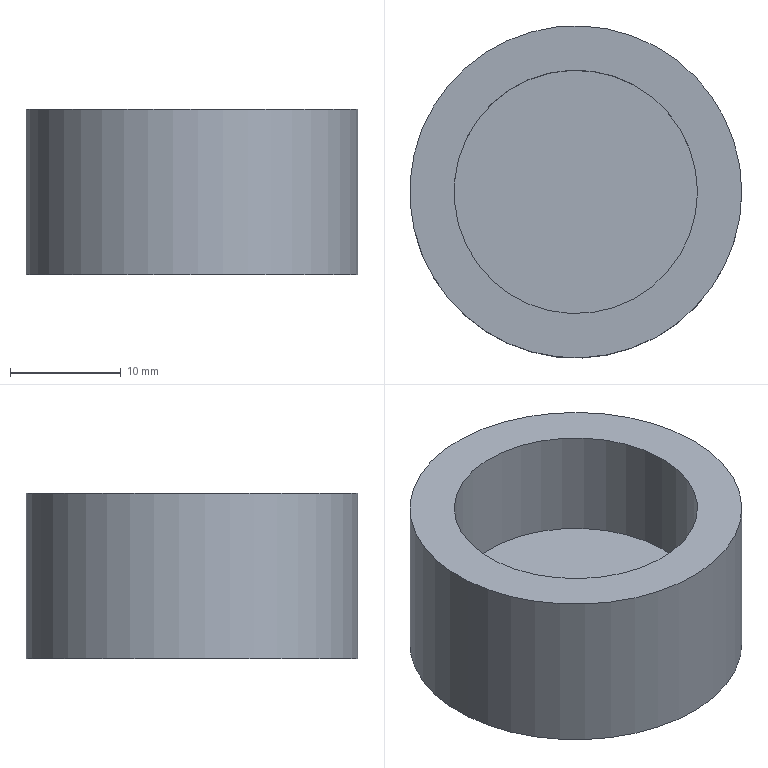Component | NX | CUP | 1 solid | 5 faces | box 30 x 30 x 15 mm | volume 6802 mm3 | plane 3 | cylinder 2 | commonest cylinder face diameters 30 x1 22 x1
STEP:
#1=CARTESIAN_POINT('',(0.,0.,0.));
#2=DIRECTION('',(0.,0.,1.));
#3=DIRECTION('',(1.,0.,0.));
#4=AXIS2_PLACEMENT_3D('',#1,#2,#3);
#5=CARTESIAN_POINT('',(23.5,0.,-28.5));
#6=VERTEX_POINT('',#5);
#7=CARTESIAN_POINT('',(12.5,0.,-28.5));
#8=DIRECTION('',(0.,0.,-1.));
#9=DIRECTION('',(1.,0.,0.));
#10=AXIS2_PLACEMENT_3D('',#7,#8,#9);
#11=CIRCLE('',#10,11.);
#12=CARTESIAN_POINT('',(12.5,0.,-28.5));
#13=DIRECTION('',(0.,0.,1.));
#14=DIRECTION('',(1.,0.,0.));
#15=AXIS2_PLACEMENT_3D('',#12,#13,#14);
#16=PLANE('',#15);
#17=CARTESIAN_POINT('',(11.,0.));
#18=CARTESIAN_POINT('',(11.,-19.053));
#19=CARTESIAN_POINT('',(-5.5,-9.526));
#20=CARTESIAN_POINT('',(-22.,-0.));
#21=CARTESIAN_POINT('',(-5.5,9.526));
#22=CARTESIAN_POINT('',(11.,19.053));
#23=CARTESIAN_POINT('',(11.,0.));
#24=(BOUNDED_CURVE()B_SPLINE_CURVE(2,(#17,#18,#19,#20,#21,#22,#23),.UNSPECIFIED.,.T.,.F.)B_SPLINE_CURVE_WITH_KNOTS((1,2,2,2,2,1),(-2.094,0.,2.094,4.189,6.283,8.378),.UNSPECIFIED.)CURVE()GEOMETRIC_REPRESENTATION_ITEM()RATIONAL_B_SPLINE_CURVE((1.,0.5,1.,0.5,1.,0.5,1.))REPRESENTATION_ITEM(''));
#25=(GEOMETRIC_REPRESENTATION_CONTEXT(2)PARAMETRIC_REPRESENTATION_CONTEXT()REPRESENTATION_CONTEXT('',''));
#26=DEFINITIONAL_REPRESENTATION('',(#24),#25);
#27=PCURVE('',#16,#26);
#28=CARTESIAN_POINT('',(12.5,0.,-38.5));
#29=DIRECTION('',(0.,0.,1.));
#30=DIRECTION('',(1.,0.,0.));
#31=AXIS2_PLACEMENT_3D('',#28,#29,#30);
#32=CYLINDRICAL_SURFACE('',#31,11.);
#33=CARTESIAN_POINT('',(6.283,10.));
#34=DIRECTION('',(-1.,0.));
#35=VECTOR('',#34,1.);
#36=LINE('',#33,#35);
#37=(GEOMETRIC_REPRESENTATION_CONTEXT(2)PARAMETRIC_REPRESENTATION_CONTEXT()REPRESENTATION_CONTEXT('',''));
#38=DEFINITIONAL_REPRESENTATION('',(#36),#37);
#39=PCURVE('',#32,#38);
#40=SURFACE_CURVE('',#11,(#27,#39),.PCURVE_S1.);
#41=EDGE_CURVE('',#6,#6,#40,.T.);
#42=ORIENTED_EDGE('',*,*,#41,.T.);
#43=EDGE_LOOP('',(#42));
#44=FACE_BOUND('',#43,.T.);
#45=CARTESIAN_POINT('',(27.5,0.,-28.5));
#46=VERTEX_POINT('',#45);
#47=CARTESIAN_POINT('',(12.5,0.,-28.5));
#48=DIRECTION('',(0.,0.,-1.));
#49=DIRECTION('',(1.,0.,0.));
#50=AXIS2_PLACEMENT_3D('',#47,#48,#49);
#51=CIRCLE('',#50,15.);
#52=CARTESIAN_POINT('',(15.,0.));
#53=CARTESIAN_POINT('',(15.,-25.981));
#54=CARTESIAN_POINT('',(-7.5,-12.99));
#55=CARTESIAN_POINT('',(-30.,-0.));
#56=CARTESIAN_POINT('',(-7.5,12.99));
#57=CARTESIAN_POINT('',(15.,25.981));
#58=CARTESIAN_POINT('',(15.,0.));
#59=(BOUNDED_CURVE()B_SPLINE_CURVE(2,(#52,#53,#54,#55,#56,#57,#58),.UNSPECIFIED.,.T.,.F.)B_SPLINE_CURVE_WITH_KNOTS((1,2,2,2,2,1),(-2.094,0.,2.094,4.189,6.283,8.378),.UNSPECIFIED.)CURVE()GEOMETRIC_REPRESENTATION_ITEM()RATIONAL_B_SPLINE_CURVE((1.,0.5,1.,0.5,1.,0.5,1.))REPRESENTATION_ITEM(''));
#60=(GEOMETRIC_REPRESENTATION_CONTEXT(2)PARAMETRIC_REPRESENTATION_CONTEXT()REPRESENTATION_CONTEXT('',''));
#61=DEFINITIONAL_REPRESENTATION('',(#59),#60);
#62=PCURVE('',#16,#61);
#63=CARTESIAN_POINT('',(12.5,0.,-43.5));
#64=DIRECTION('',(0.,0.,1.));
#65=DIRECTION('',(1.,0.,0.));
#66=AXIS2_PLACEMENT_3D('',#63,#64,#65);
#67=CYLINDRICAL_SURFACE('',#66,15.);
#68=CARTESIAN_POINT('',(6.283,15.));
#69=DIRECTION('',(-1.,0.));
#70=VECTOR('',#69,1.);
#71=LINE('',#68,#70);
#72=(GEOMETRIC_REPRESENTATION_CONTEXT(2)PARAMETRIC_REPRESENTATION_CONTEXT()REPRESENTATION_CONTEXT('',''));
#73=DEFINITIONAL_REPRESENTATION('',(#71),#72);
#74=PCURVE('',#67,#73);
#75=SURFACE_CURVE('',#51,(#62,#74),.PCURVE_S1.);
#76=EDGE_CURVE('',#46,#46,#75,.T.);
#77=ORIENTED_EDGE('',*,*,#76,.F.);
#78=EDGE_LOOP('',(#77));
#79=FACE_BOUND('',#78,.T.);
#80=ADVANCED_FACE('',(#44,#79),#16,.T.);
#81=CARTESIAN_POINT('',(27.5,0.,-43.5));
#82=VERTEX_POINT('',#81);
#83=CARTESIAN_POINT('',(12.5,0.,-43.5));
#84=DIRECTION('',(0.,0.,1.));
#85=DIRECTION('',(1.,0.,0.));
#86=AXIS2_PLACEMENT_3D('',#83,#84,#85);
#87=CIRCLE('',#86,15.);
#88=CARTESIAN_POINT('',(12.5,0.,-43.5));
#89=DIRECTION('',(0.,0.,-1.));
#90=DIRECTION('',(-1.,0.,0.));
#91=AXIS2_PLACEMENT_3D('',#88,#89,#90);
#92=PLANE('',#91);
#93=CARTESIAN_POINT('',(-15.,0.));
#94=CARTESIAN_POINT('',(-15.,25.981));
#95=CARTESIAN_POINT('',(7.5,12.99));
#96=CARTESIAN_POINT('',(30.,0.));
#97=CARTESIAN_POINT('',(7.5,-12.99));
#98=CARTESIAN_POINT('',(-15.,-25.981));
#99=CARTESIAN_POINT('',(-15.,0.));
#100=(BOUNDED_CURVE()B_SPLINE_CURVE(2,(#93,#94,#95,#96,#97,#98,#99),.UNSPECIFIED.,.T.,.F.)B_SPLINE_CURVE_WITH_KNOTS((1,2,2,2,2,1),(-2.094,0.,2.094,4.189,6.283,8.378),.UNSPECIFIED.)CURVE()GEOMETRIC_REPRESENTATION_ITEM()RATIONAL_B_SPLINE_CURVE((1.,0.5,1.,0.5,1.,0.5,1.))REPRESENTATION_ITEM(''));
#101=(GEOMETRIC_REPRESENTATION_CONTEXT(2)PARAMETRIC_REPRESENTATION_CONTEXT()REPRESENTATION_CONTEXT('',''));
#102=DEFINITIONAL_REPRESENTATION('',(#100),#101);
#103=PCURVE('',#92,#102);
#104=CARTESIAN_POINT('',(0.,0.));
#105=DIRECTION('',(1.,0.));
#106=VECTOR('',#105,1.);
#107=LINE('',#104,#106);
#108=(GEOMETRIC_REPRESENTATION_CONTEXT(2)PARAMETRIC_REPRESENTATION_CONTEXT()REPRESENTATION_CONTEXT('',''));
#109=DEFINITIONAL_REPRESENTATION('',(#107),#108);
#110=PCURVE('',#67,#109);
#111=SURFACE_CURVE('',#87,(#103,#110),.PCURVE_S1.);
#112=EDGE_CURVE('',#82,#82,#111,.T.);
#113=ORIENTED_EDGE('',*,*,#112,.F.);
#114=EDGE_LOOP('',(#113));
#115=FACE_BOUND('',#114,.T.);
#116=ADVANCED_FACE('',(#115),#92,.T.);
#117=ORIENTED_EDGE('',*,*,#76,.T.);
#118=CARTESIAN_POINT('',(27.5,-0.,-43.5));
#119=CARTESIAN_POINT('',(27.5,-0.,-28.5));
#120=B_SPLINE_CURVE_WITH_KNOTS('',1,(#118,#119),.UNSPECIFIED.,.F.,.F.,(2,2),(0.,15.),.PIECEWISE_BEZIER_KNOTS.);
#121=CARTESIAN_POINT('',(0.,0.));
#122=DIRECTION('',(0.,1.));
#123=VECTOR('',#122,1.);
#124=LINE('',#121,#123);
#125=(GEOMETRIC_REPRESENTATION_CONTEXT(2)PARAMETRIC_REPRESENTATION_CONTEXT()REPRESENTATION_CONTEXT('',''));
#126=DEFINITIONAL_REPRESENTATION('',(#124),#125);
#127=PCURVE('',#67,#126);
#128=CARTESIAN_POINT('',(6.283,0.));
#129=DIRECTION('',(0.,1.));
#130=VECTOR('',#129,1.);
#131=LINE('',#128,#130);
#132=(GEOMETRIC_REPRESENTATION_CONTEXT(2)PARAMETRIC_REPRESENTATION_CONTEXT()REPRESENTATION_CONTEXT('',''));
#133=DEFINITIONAL_REPRESENTATION('',(#131),#132);
#134=PCURVE('',#67,#133);
#135=SEAM_CURVE('',#120,(#127,#134),.PCURVE_S1.);
#136=EDGE_CURVE('',#82,#46,#135,.T.);
#137=ORIENTED_EDGE('',*,*,#136,.F.);
#138=ORIENTED_EDGE('',*,*,#112,.T.);
#139=ORIENTED_EDGE('',*,*,#136,.T.);
#140=EDGE_LOOP('',(#117,#137,#138,#139));
#141=FACE_BOUND('',#140,.T.);
#142=ADVANCED_FACE('',(#141),#67,.T.);
#143=CARTESIAN_POINT('',(23.5,0.,-38.5));
#144=VERTEX_POINT('',#143);
#145=CARTESIAN_POINT('',(12.5,0.,-38.5));
#146=DIRECTION('',(0.,0.,1.));
#147=DIRECTION('',(1.,0.,0.));
#148=AXIS2_PLACEMENT_3D('',#145,#146,#147);
#149=CIRCLE('',#148,11.);
#150=CARTESIAN_POINT('',(0.,0.));
#151=DIRECTION('',(1.,0.));
#152=VECTOR('',#151,1.);
#153=LINE('',#150,#152);
#154=(GEOMETRIC_REPRESENTATION_CONTEXT(2)PARAMETRIC_REPRESENTATION_CONTEXT()REPRESENTATION_CONTEXT('',''));
#155=DEFINITIONAL_REPRESENTATION('',(#153),#154);
#156=PCURVE('',#32,#155);
#157=CARTESIAN_POINT('',(12.5,0.,-38.5));
#158=DIRECTION('',(0.,0.,-1.));
#159=DIRECTION('',(-1.,0.,0.));
#160=AXIS2_PLACEMENT_3D('',#157,#158,#159);
#161=PLANE('',#160);
#162=CARTESIAN_POINT('',(-11.,0.));
#163=CARTESIAN_POINT('',(-11.,19.053));
#164=CARTESIAN_POINT('',(5.5,9.526));
#165=CARTESIAN_POINT('',(22.,0.));
#166=CARTESIAN_POINT('',(5.5,-9.526));
#167=CARTESIAN_POINT('',(-11.,-19.053));
#168=CARTESIAN_POINT('',(-11.,0.));
#169=(BOUNDED_CURVE()B_SPLINE_CURVE(2,(#162,#163,#164,#165,#166,#167,#168),.UNSPECIFIED.,.T.,.F.)B_SPLINE_CURVE_WITH_KNOTS((1,2,2,2,2,1),(-2.094,0.,2.094,4.189,6.283,8.378),.UNSPECIFIED.)CURVE()GEOMETRIC_REPRESENTATION_ITEM()RATIONAL_B_SPLINE_CURVE((1.,0.5,1.,0.5,1.,0.5,1.))REPRESENTATION_ITEM(''));
#170=(GEOMETRIC_REPRESENTATION_CONTEXT(2)PARAMETRIC_REPRESENTATION_CONTEXT()REPRESENTATION_CONTEXT('',''));
#171=DEFINITIONAL_REPRESENTATION('',(#169),#170);
#172=PCURVE('',#161,#171);
#173=SURFACE_CURVE('',#149,(#156,#172),.PCURVE_S1.);
#174=EDGE_CURVE('',#144,#144,#173,.T.);
#175=ORIENTED_EDGE('',*,*,#174,.T.);
#176=CARTESIAN_POINT('',(23.5,0.,-38.5));
#177=CARTESIAN_POINT('',(23.5,0.,-28.5));
#178=B_SPLINE_CURVE_WITH_KNOTS('',1,(#176,#177),.UNSPECIFIED.,.F.,.F.,(2,2),(0.,10.),.PIECEWISE_BEZIER_KNOTS.);
#179=CARTESIAN_POINT('',(6.283,0.));
#180=DIRECTION('',(0.,1.));
#181=VECTOR('',#180,1.);
#182=LINE('',#179,#181);
#183=(GEOMETRIC_REPRESENTATION_CONTEXT(2)PARAMETRIC_REPRESENTATION_CONTEXT()REPRESENTATION_CONTEXT('',''));
#184=DEFINITIONAL_REPRESENTATION('',(#182),#183);
#185=PCURVE('',#32,#184);
#186=CARTESIAN_POINT('',(0.,0.));
#187=DIRECTION('',(0.,1.));
#188=VECTOR('',#187,1.);
#189=LINE('',#186,#188);
#190=(GEOMETRIC_REPRESENTATION_CONTEXT(2)PARAMETRIC_REPRESENTATION_CONTEXT()REPRESENTATION_CONTEXT('',''));
#191=DEFINITIONAL_REPRESENTATION('',(#189),#190);
#192=PCURVE('',#32,#191);
#193=SEAM_CURVE('',#178,(#185,#192),.PCURVE_S1.);
#194=EDGE_CURVE('',#144,#6,#193,.T.);
#195=ORIENTED_EDGE('',*,*,#194,.T.);
#196=ORIENTED_EDGE('',*,*,#41,.T.);
#197=ORIENTED_EDGE('',*,*,#194,.F.);
#198=EDGE_LOOP('',(#175,#195,#196,#197));
#199=FACE_BOUND('',#198,.F.);
#200=ADVANCED_FACE('',(#199),#32,.F.);
#201=ORIENTED_EDGE('',*,*,#174,.T.);
#202=EDGE_LOOP('',(#201));
#203=FACE_BOUND('',#202,.T.);
#204=ADVANCED_FACE('',(#203),#161,.F.);
#205=CLOSED_SHELL('',(#80,#116,#142,#200,#204));
#206=MANIFOLD_SOLID_BREP('',#205);
#207=(LENGTH_UNIT()NAMED_UNIT(*)SI_UNIT(.MILLI.,.METRE.));
#208=UNCERTAINTY_MEASURE_WITH_UNIT(LENGTH_MEASURE(0.00001),#207,'','');
#209=(NAMED_UNIT(*)PLANE_ANGLE_UNIT()SI_UNIT($,.RADIAN.));
#210=(NAMED_UNIT(*)SI_UNIT($,.STERADIAN.)SOLID_ANGLE_UNIT());
#211=(GEOMETRIC_REPRESENTATION_CONTEXT(3)GLOBAL_UNCERTAINTY_ASSIGNED_CONTEXT((#208))GLOBAL_UNIT_ASSIGNED_CONTEXT((#207,#209,#210))REPRESENTATION_CONTEXT('',''));
#212=ADVANCED_BREP_SHAPE_REPRESENTATION('',(#4,#206),#211);